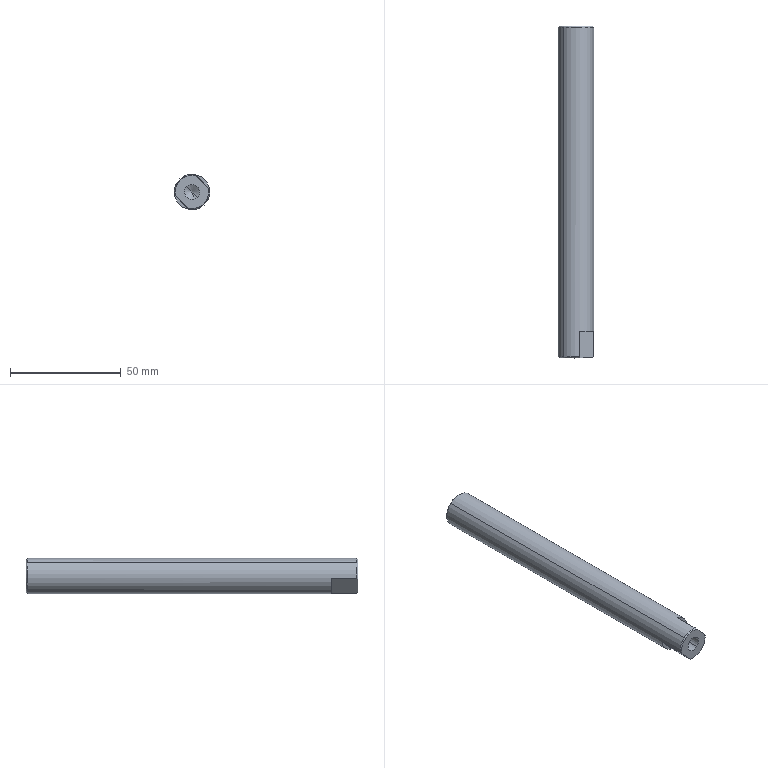Component | SolidWorks | SL021-102-4065.SL4PRT-5 | 1 solid | 21 faces | box 16 x 150 x 16 mm | volume 27965 mm3 | cone 9 | cylinder 6 | plane 6 | commonest cylinder face diameters 6.8 x4 16 x2 | material Bearing Steel
build123d program:
from build123d import *

# Parameters (mm, degrees)
SKETCH1_R           = 8
BOSS_EXTRUDE1_DEPTH = 75
CHAMFER1_SIZE       = 0.5
SKETCH4_OUTSIDE_W   = 48.34
SKETCH4_OUTSIDE_H   = 48.34
SKETCH4_OUTSIDE_W_2 = 13
SKETCH4_OUTSIDE_H_2 = 21.2
CUT_EXTRUDE1_DEPTH  = 12


with BuildPart() as part:
    # Sketch1 → Boss-Extrude1 (new, symmetric)
    with BuildSketch(Plane(origin=(0, 0, 0), x_dir=(1, 0, 0), z_dir=(0, 1, 0))):
        with Locations(Location((0, 0, 0), (0, 0, 270))):
            Circle(SKETCH1_R)
    extrude(amount=BOSS_EXTRUDE1_DEPTH, both=True)

    # Chamfer1
    chamfer1_edges = [part.edges().sort_by_distance(p)[0] for p in [
        (0, -75, -8),
        (0, 75, -8),
    ]]
    chamfer(chamfer1_edges, length=CHAMFER1_SIZE)

    # Sketch2 → M8 Tapped Hole1 (revolve, cut)
    with BuildSketch(Plane(origin=(0, 75, 0), x_dir=(0, 0, 1), z_dir=(1, 0, 0))):
        Polygon((0, 0), (0, 28.293), (3.4, 26.25), (3.4, 0), align=None)
    m8_tapped_hole1 = revolve(axis=Axis((0, 81.35, 0), (0, -1, 0)), mode=Mode.SUBTRACT)

    # Mirror1: M8 Tapped Hole1 across plane
    add(m8_tapped_hole1.mirror(Plane.ZX), mode=Mode.SUBTRACT)

    # Sketch4 outside → Cut-Extrude1 (cut)
    with BuildSketch(Plane.XZ.offset(75)):
        Rectangle(SKETCH4_OUTSIDE_W, SKETCH4_OUTSIDE_H)
        Rectangle(SKETCH4_OUTSIDE_W_2, SKETCH4_OUTSIDE_H_2, mode=Mode.SUBTRACT)
    extrude(amount=-CUT_EXTRUDE1_DEPTH, mode=Mode.SUBTRACT)


solid = part.part

# Placed as in the assembly
solid = solid.moved(Location((-126.163, -15.499, -306.378), (180, 42.687, -180)))
STEP:
#1=COLOUR_RGB('',0.7922,0.8196,0.9333);
#2=FILL_AREA_STYLE_COLOUR('',#1);
#3=FILL_AREA_STYLE('',(#2));
#4=SURFACE_STYLE_FILL_AREA(#3);
#5=SURFACE_SIDE_STYLE('',(#4));
#6=SURFACE_STYLE_USAGE(.BOTH.,#5);
#7=PRESENTATION_STYLE_ASSIGNMENT((#6));
#8=CARTESIAN_POINT('',(-4.876,-2.529,-12.161));
#9=VERTEX_POINT('',#8);
#10=CARTESIAN_POINT('',(-5.058,-2.529,-11.964));
#11=VERTEX_POINT('',#10);
#12=CARTESIAN_POINT('',(-4.967,-2.529,-12.062));
#13=DIRECTION('',(0.,-1.,0.));
#14=DIRECTION('',(-0.678,0.,0.7351));
#15=AXIS2_PLACEMENT_3D('',#12,#13,#14);
#16=CIRCLE('',#15,0.1339);
#17=EDGE_CURVE('',#9,#11,#16,.T.);
#18=ORIENTED_EDGE('',*,*,#17,.F.);
#19=CARTESIAN_POINT('',(-4.876,-3.563,-12.161));
#20=VERTEX_POINT('',#19);
#21=CARTESIAN_POINT('',(-4.876,-3.563,-12.161));
#22=DIRECTION('',(0.,-1.,0.));
#23=VECTOR('',#22,39.37);
#24=LINE('',#21,#23);
#25=EDGE_CURVE('',#9,#20,#24,.T.);
#26=ORIENTED_EDGE('',*,*,#25,.T.);
#27=CARTESIAN_POINT('',(-5.058,-3.563,-11.964));
#28=VERTEX_POINT('',#27);
#29=CARTESIAN_POINT('',(-4.967,-3.563,-12.062));
#30=DIRECTION('',(0.,-1.,0.));
#31=DIRECTION('',(-0.678,0.,0.7351));
#32=AXIS2_PLACEMENT_3D('',#29,#30,#31);
#33=CIRCLE('',#32,0.1339);
#34=EDGE_CURVE('',#20,#28,#33,.T.);
#35=ORIENTED_EDGE('',*,*,#34,.T.);
#36=CARTESIAN_POINT('',(-5.058,-3.563,-11.964));
#37=DIRECTION('',(0.,-1.,0.));
#38=VECTOR('',#37,39.37);
#39=LINE('',#36,#38);
#40=EDGE_CURVE('',#11,#28,#39,.T.);
#41=ORIENTED_EDGE('',*,*,#40,.F.);
#42=EDGE_LOOP('',(#18,#26,#35,#41));
#43=FACE_OUTER_BOUND('',#42,.T.);
#44=CARTESIAN_POINT('',(-4.967,-3.563,-12.062));
#45=DIRECTION('',(0.,-1.,0.));
#46=DIRECTION('',(-0.678,0.,0.7351));
#47=AXIS2_PLACEMENT_3D('',#44,#45,#46);
#48=CYLINDRICAL_SURFACE('',#47,0.1339);
#49=ADVANCED_FACE('',(#43),#48,.F.);
#50=CARTESIAN_POINT('',(-4.967,-2.449,-12.062));
#51=VERTEX_POINT('',#50);
#52=CARTESIAN_POINT('',(-5.058,-2.529,-11.964));
#53=DIRECTION('',(-0.5811,-0.515,0.6301));
#54=VECTOR('',#53,39.37);
#55=LINE('',#52,#54);
#56=EDGE_CURVE('',#51,#11,#55,.T.);
#57=ORIENTED_EDGE('',*,*,#56,.F.);
#58=CARTESIAN_POINT('',(-4.876,-2.529,-12.161));
#59=DIRECTION('',(0.5811,-0.515,-0.6301));
#60=VECTOR('',#59,39.37);
#61=LINE('',#58,#60);
#62=EDGE_CURVE('',#51,#9,#61,.T.);
#63=ORIENTED_EDGE('',*,*,#62,.T.);
#64=ORIENTED_EDGE('',*,*,#17,.T.);
#65=EDGE_LOOP('',(#57,#63,#64));
#66=FACE_OUTER_BOUND('',#65,.T.);
#67=CARTESIAN_POINT('',(-4.967,-2.529,-12.062));
#68=DIRECTION('',(0.,-1.,0.));
#69=DIRECTION('',(-0.678,0.,0.7351));
#70=AXIS2_PLACEMENT_3D('',#67,#68,#69);
#71=CONICAL_SURFACE('',#70,0.1339,1.03);
#72=ADVANCED_FACE('',(#66),#71,.F.);
#73=CARTESIAN_POINT('',(-5.058,1.309,-11.964));
#74=VERTEX_POINT('',#73);
#75=CARTESIAN_POINT('',(-4.876,1.309,-12.161));
#76=VERTEX_POINT('',#75);
#77=CARTESIAN_POINT('',(-4.967,1.309,-12.062));
#78=DIRECTION('',(-0.,1.,-0.));
#79=DIRECTION('',(0.678,0.,-0.7351));
#80=AXIS2_PLACEMENT_3D('',#77,#78,#79);
#81=CIRCLE('',#80,0.1339);
#82=EDGE_CURVE('',#74,#76,#81,.T.);
#83=ORIENTED_EDGE('',*,*,#82,.F.);
#84=CARTESIAN_POINT('',(-5.058,2.343,-11.964));
#85=VERTEX_POINT('',#84);
#86=CARTESIAN_POINT('',(-5.058,2.343,-11.964));
#87=DIRECTION('',(-0.,1.,-0.));
#88=VECTOR('',#87,39.37);
#89=LINE('',#86,#88);
#90=EDGE_CURVE('',#74,#85,#89,.T.);
#91=ORIENTED_EDGE('',*,*,#90,.T.);
#92=CARTESIAN_POINT('',(-4.876,2.343,-12.161));
#93=VERTEX_POINT('',#92);
#94=CARTESIAN_POINT('',(-4.967,2.343,-12.062));
#95=DIRECTION('',(-0.,1.,-0.));
#96=DIRECTION('',(0.678,0.,-0.7351));
#97=AXIS2_PLACEMENT_3D('',#94,#95,#96);
#98=CIRCLE('',#97,0.1339);
#99=EDGE_CURVE('',#85,#93,#98,.T.);
#100=ORIENTED_EDGE('',*,*,#99,.T.);
#101=CARTESIAN_POINT('',(-4.876,2.343,-12.161));
#102=DIRECTION('',(-0.,1.,-0.));
#103=VECTOR('',#102,39.37);
#104=LINE('',#101,#103);
#105=EDGE_CURVE('',#76,#93,#104,.T.);
#106=ORIENTED_EDGE('',*,*,#105,.F.);
#107=EDGE_LOOP('',(#83,#91,#100,#106));
#108=FACE_OUTER_BOUND('',#107,.T.);
#109=CARTESIAN_POINT('',(-4.967,2.343,-12.062));
#110=DIRECTION('',(-0.,1.,-0.));
#111=DIRECTION('',(0.678,0.,-0.7351));
#112=AXIS2_PLACEMENT_3D('',#109,#110,#111);
#113=CYLINDRICAL_SURFACE('',#112,0.1339);
#114=ADVANCED_FACE('',(#108),#113,.F.);
#115=CARTESIAN_POINT('',(-4.967,1.229,-12.062));
#116=VERTEX_POINT('',#115);
#117=CARTESIAN_POINT('',(-4.876,1.309,-12.161));
#118=DIRECTION('',(0.5811,0.515,-0.6301));
#119=VECTOR('',#118,39.37);
#120=LINE('',#117,#119);
#121=EDGE_CURVE('',#116,#76,#120,.T.);
#122=ORIENTED_EDGE('',*,*,#121,.F.);
#123=CARTESIAN_POINT('',(-5.058,1.309,-11.964));
#124=DIRECTION('',(-0.5811,0.515,0.6301));
#125=VECTOR('',#124,39.37);
#126=LINE('',#123,#125);
#127=EDGE_CURVE('',#116,#74,#126,.T.);
#128=ORIENTED_EDGE('',*,*,#127,.T.);
#129=ORIENTED_EDGE('',*,*,#82,.T.);
#130=EDGE_LOOP('',(#122,#128,#129));
#131=FACE_OUTER_BOUND('',#130,.T.);
#132=CARTESIAN_POINT('',(-4.967,1.309,-12.062));
#133=DIRECTION('',(-0.,1.,-0.));
#134=DIRECTION('',(0.678,0.,-0.7351));
#135=AXIS2_PLACEMENT_3D('',#132,#133,#134);
#136=CONICAL_SURFACE('',#135,0.1339,1.03);
#137=ADVANCED_FACE('',(#131),#136,.F.);
#138=CARTESIAN_POINT('',(-4.767,2.343,-12.279));
#139=VERTEX_POINT('',#138);
#140=CARTESIAN_POINT('',(-5.167,2.343,-11.845));
#141=VERTEX_POINT('',#140);
#142=CARTESIAN_POINT('',(-4.967,2.343,-12.062));
#143=DIRECTION('',(-0.,1.,-0.));
#144=DIRECTION('',(0.678,0.,-0.7351));
#145=AXIS2_PLACEMENT_3D('',#142,#143,#144);
#146=CIRCLE('',#145,0.2953);
#147=EDGE_CURVE('',#139,#141,#146,.T.);
#148=ORIENTED_EDGE('',*,*,#147,.F.);
#149=CARTESIAN_POINT('',(-4.754,2.323,-12.294));
#150=VERTEX_POINT('',#149);
#151=CARTESIAN_POINT('',(-4.767,2.343,-12.279));
#152=DIRECTION('',(0.4794,-0.7071,-0.5198));
#153=VECTOR('',#152,39.37);
#154=LINE('',#151,#153);
#155=EDGE_CURVE('',#139,#150,#154,.T.);
#156=ORIENTED_EDGE('',*,*,#155,.T.);
#157=CARTESIAN_POINT('',(-5.181,2.323,-11.831));
#158=VERTEX_POINT('',#157);
#159=CARTESIAN_POINT('',(-4.967,2.323,-12.062));
#160=DIRECTION('',(0.,-1.,0.));
#161=DIRECTION('',(0.678,0.,-0.7351));
#162=AXIS2_PLACEMENT_3D('',#159,#160,#161);
#163=CIRCLE('',#162,0.315);
#164=EDGE_CURVE('',#158,#150,#163,.T.);
#165=ORIENTED_EDGE('',*,*,#164,.F.);
#166=CARTESIAN_POINT('',(-5.167,2.343,-11.845));
#167=DIRECTION('',(-0.4794,-0.7071,0.5198));
#168=VECTOR('',#167,39.37);
#169=LINE('',#166,#168);
#170=EDGE_CURVE('',#141,#158,#169,.T.);
#171=ORIENTED_EDGE('',*,*,#170,.F.);
#172=EDGE_LOOP('',(#148,#156,#165,#171));
#173=FACE_OUTER_BOUND('',#172,.T.);
#174=CARTESIAN_POINT('',(-4.967,2.343,-12.062));
#175=DIRECTION('',(0.,-1.,0.));
#176=DIRECTION('',(-0.678,0.,0.7351));
#177=AXIS2_PLACEMENT_3D('',#174,#175,#176);
#178=CONICAL_SURFACE('',#177,0.2953,0.7854);
#179=ADVANCED_FACE('',(#173),#178,.T.);
#180=CARTESIAN_POINT('',(-4.767,-3.563,-12.279));
#181=VERTEX_POINT('',#180);
#182=CARTESIAN_POINT('',(-4.679,-3.563,-11.997));
#183=VERTEX_POINT('',#182);
#184=CARTESIAN_POINT('',(-4.967,-3.563,-12.062));
#185=DIRECTION('',(0.,-1.,0.));
#186=DIRECTION('',(0.678,0.,-0.7351));
#187=AXIS2_PLACEMENT_3D('',#184,#185,#186);
#188=CIRCLE('',#187,0.2953);
#189=EDGE_CURVE('',#181,#183,#188,.T.);
#190=ORIENTED_EDGE('',*,*,#189,.F.);
#191=CARTESIAN_POINT('',(-4.754,-3.543,-12.294));
#192=VERTEX_POINT('',#191);
#193=CARTESIAN_POINT('',(-4.754,-3.543,-12.294));
#194=DIRECTION('',(0.4794,0.7071,-0.5198));
#195=VECTOR('',#194,39.37);
#196=LINE('',#193,#195);
#197=EDGE_CURVE('',#181,#192,#196,.T.);
#198=ORIENTED_EDGE('',*,*,#197,.T.);
#199=CARTESIAN_POINT('',(-4.654,-3.543,-12.024));
#200=VERTEX_POINT('',#199);
#201=CARTESIAN_POINT('',(-4.967,-3.543,-12.062));
#202=DIRECTION('',(-0.,1.,-0.));
#203=DIRECTION('',(0.678,0.,-0.7351));
#204=AXIS2_PLACEMENT_3D('',#201,#202,#203);
#205=CIRCLE('',#204,0.315);
#206=EDGE_CURVE('',#200,#192,#205,.T.);
#207=ORIENTED_EDGE('',*,*,#206,.F.);
#208=CARTESIAN_POINT('',(-4.654,-3.543,-12.024));
#209=CARTESIAN_POINT('',(-4.663,-3.55,-12.015));
#210=CARTESIAN_POINT('',(-4.671,-3.557,-12.006));
#211=CARTESIAN_POINT('',(-4.679,-3.563,-11.997));
#212=B_SPLINE_CURVE_WITH_KNOTS('',3,(#208,#209,#210,#211),.UNSPECIFIED.,.F.,.F.,(4,4),(0.01516,0.01621),.UNSPECIFIED.);
#213=EDGE_CURVE('',#200,#183,#212,.T.);
#214=ORIENTED_EDGE('',*,*,#213,.T.);
#215=EDGE_LOOP('',(#190,#198,#207,#214));
#216=FACE_OUTER_BOUND('',#215,.T.);
#217=CARTESIAN_POINT('',(-4.967,-3.543,-12.062));
#218=DIRECTION('',(-0.,1.,-0.));
#219=DIRECTION('',(0.678,0.,-0.7351));
#220=AXIS2_PLACEMENT_3D('',#217,#218,#219);
#221=CONICAL_SURFACE('',#220,0.315,0.7854);
#222=ADVANCED_FACE('',(#216),#221,.T.);
#223=ORIENTED_EDGE('',*,*,#164,.T.);
#224=CARTESIAN_POINT('',(-4.754,2.343,-12.294));
#225=DIRECTION('',(0.,-1.,0.));
#226=VECTOR('',#225,39.37);
#227=LINE('',#224,#226);
#228=EDGE_CURVE('',#150,#192,#227,.T.);
#229=ORIENTED_EDGE('',*,*,#228,.T.);
#230=CARTESIAN_POINT('',(-5.031,-3.543,-12.371));
#231=VERTEX_POINT('',#230);
#232=CARTESIAN_POINT('',(-4.967,-3.543,-12.062));
#233=DIRECTION('',(-0.,1.,-0.));
#234=DIRECTION('',(0.678,0.,-0.7351));
#235=AXIS2_PLACEMENT_3D('',#232,#233,#234);
#236=CIRCLE('',#235,0.315);
#237=EDGE_CURVE('',#192,#231,#236,.T.);
#238=ORIENTED_EDGE('',*,*,#237,.T.);
#239=CARTESIAN_POINT('',(-5.031,-3.091,-12.371));
#240=VERTEX_POINT('',#239);
#241=CARTESIAN_POINT('',(-5.031,2.343,-12.371));
#242=DIRECTION('',(0.,-1.,0.));
#243=VECTOR('',#242,39.37);
#244=LINE('',#241,#243);
#245=EDGE_CURVE('',#240,#231,#244,.T.);
#246=ORIENTED_EDGE('',*,*,#245,.F.);
#247=CARTESIAN_POINT('',(-5.28,-3.091,-12.101));
#248=VERTEX_POINT('',#247);
#249=CARTESIAN_POINT('',(-4.967,-3.091,-12.062));
#250=DIRECTION('',(0.,-1.,0.));
#251=DIRECTION('',(-0.678,0.,0.7351));
#252=AXIS2_PLACEMENT_3D('',#249,#250,#251);
#253=CIRCLE('',#252,0.315);
#254=EDGE_CURVE('',#248,#240,#253,.T.);
#255=ORIENTED_EDGE('',*,*,#254,.F.);
#256=CARTESIAN_POINT('',(-5.28,-3.543,-12.101));
#257=VERTEX_POINT('',#256);
#258=CARTESIAN_POINT('',(-5.28,2.343,-12.101));
#259=DIRECTION('',(-0.,1.,-0.));
#260=VECTOR('',#259,39.37);
#261=LINE('',#258,#260);
#262=EDGE_CURVE('',#257,#248,#261,.T.);
#263=ORIENTED_EDGE('',*,*,#262,.F.);
#264=CARTESIAN_POINT('',(-5.181,-3.543,-11.831));
#265=VERTEX_POINT('',#264);
#266=CARTESIAN_POINT('',(-4.967,-3.543,-12.062));
#267=DIRECTION('',(-0.,1.,-0.));
#268=DIRECTION('',(0.678,0.,-0.7351));
#269=AXIS2_PLACEMENT_3D('',#266,#267,#268);
#270=CIRCLE('',#269,0.315);
#271=EDGE_CURVE('',#257,#265,#270,.T.);
#272=ORIENTED_EDGE('',*,*,#271,.T.);
#273=CARTESIAN_POINT('',(-5.181,2.343,-11.831));
#274=DIRECTION('',(0.,-1.,0.));
#275=VECTOR('',#274,39.37);
#276=LINE('',#273,#275);
#277=EDGE_CURVE('',#158,#265,#276,.T.);
#278=ORIENTED_EDGE('',*,*,#277,.F.);
#279=EDGE_LOOP('',(#223,#229,#238,#246,#255,#263,#272,#278));
#280=FACE_OUTER_BOUND('',#279,.T.);
#281=CARTESIAN_POINT('',(-4.967,2.343,-12.062));
#282=DIRECTION('',(0.,-1.,0.));
#283=DIRECTION('',(-0.678,0.,0.7351));
#284=AXIS2_PLACEMENT_3D('',#281,#282,#283);
#285=CYLINDRICAL_SURFACE('',#284,0.315);
#286=ADVANCED_FACE('',(#280),#285,.T.);
#287=ORIENTED_EDGE('',*,*,#228,.F.);
#288=CARTESIAN_POINT('',(-4.967,2.323,-12.062));
#289=DIRECTION('',(0.,-1.,0.));
#290=DIRECTION('',(0.678,0.,-0.7351));
#291=AXIS2_PLACEMENT_3D('',#288,#289,#290);
#292=CIRCLE('',#291,0.315);
#293=EDGE_CURVE('',#150,#158,#292,.T.);
#294=ORIENTED_EDGE('',*,*,#293,.T.);
#295=ORIENTED_EDGE('',*,*,#277,.T.);
#296=CARTESIAN_POINT('',(-4.903,-3.543,-11.754));
#297=VERTEX_POINT('',#296);
#298=CARTESIAN_POINT('',(-4.967,-3.543,-12.062));
#299=DIRECTION('',(-0.,1.,-0.));
#300=DIRECTION('',(0.678,0.,-0.7351));
#301=AXIS2_PLACEMENT_3D('',#298,#299,#300);
#302=CIRCLE('',#301,0.315);
#303=EDGE_CURVE('',#265,#297,#302,.T.);
#304=ORIENTED_EDGE('',*,*,#303,.T.);
#305=CARTESIAN_POINT('',(-4.903,-3.091,-11.754));
#306=VERTEX_POINT('',#305);
#307=CARTESIAN_POINT('',(-4.903,2.343,-11.754));
#308=DIRECTION('',(0.,-1.,0.));
#309=VECTOR('',#308,39.37);
#310=LINE('',#307,#309);
#311=EDGE_CURVE('',#306,#297,#310,.T.);
#312=ORIENTED_EDGE('',*,*,#311,.F.);
#313=CARTESIAN_POINT('',(-4.654,-3.091,-12.024));
#314=VERTEX_POINT('',#313);
#315=CARTESIAN_POINT('',(-4.967,-3.091,-12.062));
#316=DIRECTION('',(0.,-1.,0.));
#317=DIRECTION('',(-0.678,0.,0.7351));
#318=AXIS2_PLACEMENT_3D('',#315,#316,#317);
#319=CIRCLE('',#318,0.315);
#320=EDGE_CURVE('',#314,#306,#319,.T.);
#321=ORIENTED_EDGE('',*,*,#320,.F.);
#322=CARTESIAN_POINT('',(-4.654,2.343,-12.024));
#323=DIRECTION('',(-0.,1.,-0.));
#324=VECTOR('',#323,39.37);
#325=LINE('',#322,#324);
#326=EDGE_CURVE('',#200,#314,#325,.T.);
#327=ORIENTED_EDGE('',*,*,#326,.F.);
#328=ORIENTED_EDGE('',*,*,#206,.T.);
#329=EDGE_LOOP('',(#287,#294,#295,#304,#312,#321,#327,#328));
#330=FACE_OUTER_BOUND('',#329,.T.);
#331=CARTESIAN_POINT('',(-4.967,2.343,-12.062));
#332=DIRECTION('',(0.,-1.,0.));
#333=DIRECTION('',(-0.678,0.,0.7351));
#334=AXIS2_PLACEMENT_3D('',#331,#332,#333);
#335=CYLINDRICAL_SURFACE('',#334,0.315);
#336=ADVANCED_FACE('',(#330),#335,.T.);
#337=CARTESIAN_POINT('',(-4.967,-3.563,-12.062));
#338=DIRECTION('',(0.,-1.,0.));
#339=DIRECTION('',(-0.678,0.,0.7351));
#340=AXIS2_PLACEMENT_3D('',#337,#338,#339);
#341=CIRCLE('',#340,0.1339);
#342=EDGE_CURVE('',#28,#20,#341,.T.);
#343=ORIENTED_EDGE('',*,*,#342,.F.);
#344=ORIENTED_EDGE('',*,*,#34,.F.);
#345=EDGE_LOOP('',(#343,#344));
#346=FACE_BOUND('',#345,.T.);
#347=CARTESIAN_POINT('',(-5.255,-3.563,-12.127));
#348=VERTEX_POINT('',#347);
#349=CARTESIAN_POINT('',(-5.055,-3.563,-12.344));
#350=VERTEX_POINT('',#349);
#351=CARTESIAN_POINT('',(-5.438,-3.563,-11.929));
#352=DIRECTION('',(0.678,-0.,-0.7351));
#353=VECTOR('',#352,39.37);
#354=LINE('',#351,#353);
#355=EDGE_CURVE('',#348,#350,#354,.T.);
#356=ORIENTED_EDGE('',*,*,#355,.T.);
#357=CARTESIAN_POINT('',(-4.967,-3.563,-12.062));
#358=DIRECTION('',(0.,-1.,0.));
#359=DIRECTION('',(0.678,0.,-0.7351));
#360=AXIS2_PLACEMENT_3D('',#357,#358,#359);
#361=CIRCLE('',#360,0.2953);
#362=EDGE_CURVE('',#350,#181,#361,.T.);
#363=ORIENTED_EDGE('',*,*,#362,.T.);
#364=ORIENTED_EDGE('',*,*,#189,.T.);
#365=CARTESIAN_POINT('',(-4.879,-3.563,-11.78));
#366=VERTEX_POINT('',#365);
#367=CARTESIAN_POINT('',(-5.062,-3.563,-11.582));
#368=DIRECTION('',(-0.678,0.,0.7351));
#369=VECTOR('',#368,39.37);
#370=LINE('',#367,#369);
#371=EDGE_CURVE('',#183,#366,#370,.T.);
#372=ORIENTED_EDGE('',*,*,#371,.T.);
#373=CARTESIAN_POINT('',(-4.967,-3.563,-12.062));
#374=DIRECTION('',(0.,-1.,0.));
#375=DIRECTION('',(0.678,0.,-0.7351));
#376=AXIS2_PLACEMENT_3D('',#373,#374,#375);
#377=CIRCLE('',#376,0.2953);
#378=EDGE_CURVE('',#366,#348,#377,.T.);
#379=ORIENTED_EDGE('',*,*,#378,.T.);
#380=EDGE_LOOP('',(#356,#363,#364,#372,#379));
#381=FACE_OUTER_BOUND('',#380,.T.);
#382=CARTESIAN_POINT('',(-4.967,-3.563,-12.062));
#383=DIRECTION('',(-0.,1.,-0.));
#384=DIRECTION('',(0.678,-0.,-0.7351));
#385=AXIS2_PLACEMENT_3D('',#382,#383,#384);
#386=PLANE('',#385);
#387=ADVANCED_FACE('',(#346,#381),#386,.F.);
#388=ORIENTED_EDGE('',*,*,#271,.F.);
#389=CARTESIAN_POINT('',(-5.28,-3.543,-12.101));
#390=CARTESIAN_POINT('',(-5.272,-3.55,-12.109));
#391=CARTESIAN_POINT('',(-5.263,-3.557,-12.118));
#392=CARTESIAN_POINT('',(-5.255,-3.563,-12.127));
#393=B_SPLINE_CURVE_WITH_KNOTS('',3,(#389,#390,#391,#392),.UNSPECIFIED.,.F.,.F.,(4,4),(0.01516,0.01621),.UNSPECIFIED.);
#394=EDGE_CURVE('',#257,#348,#393,.T.);
#395=ORIENTED_EDGE('',*,*,#394,.T.);
#396=ORIENTED_EDGE('',*,*,#378,.F.);
#397=CARTESIAN_POINT('',(-4.879,-3.563,-11.78));
#398=CARTESIAN_POINT('',(-4.887,-3.557,-11.771));
#399=CARTESIAN_POINT('',(-4.895,-3.55,-11.762));
#400=CARTESIAN_POINT('',(-4.903,-3.543,-11.754));
#401=B_SPLINE_CURVE_WITH_KNOTS('',3,(#397,#398,#399,#400),.UNSPECIFIED.,.F.,.F.,(4,4),(0.02403,0.02509),.UNSPECIFIED.);
#402=EDGE_CURVE('',#366,#297,#401,.T.);
#403=ORIENTED_EDGE('',*,*,#402,.T.);
#404=ORIENTED_EDGE('',*,*,#303,.F.);
#405=EDGE_LOOP('',(#388,#395,#396,#403,#404));
#406=FACE_OUTER_BOUND('',#405,.T.);
#407=CARTESIAN_POINT('',(-4.967,-3.543,-12.062));
#408=DIRECTION('',(-0.,1.,-0.));
#409=DIRECTION('',(0.678,0.,-0.7351));
#410=AXIS2_PLACEMENT_3D('',#407,#408,#409);
#411=CONICAL_SURFACE('',#410,0.315,0.7854);
#412=ADVANCED_FACE('',(#406),#411,.T.);
#413=ORIENTED_EDGE('',*,*,#197,.F.);
#414=ORIENTED_EDGE('',*,*,#362,.F.);
#415=CARTESIAN_POINT('',(-5.055,-3.563,-12.344));
#416=CARTESIAN_POINT('',(-5.047,-3.557,-12.353));
#417=CARTESIAN_POINT('',(-5.039,-3.55,-12.362));
#418=CARTESIAN_POINT('',(-5.031,-3.543,-12.371));
#419=B_SPLINE_CURVE_WITH_KNOTS('',3,(#415,#416,#417,#418),.UNSPECIFIED.,.F.,.F.,(4,4),(0.02403,0.02509),.UNSPECIFIED.);
#420=EDGE_CURVE('',#350,#231,#419,.T.);
#421=ORIENTED_EDGE('',*,*,#420,.T.);
#422=ORIENTED_EDGE('',*,*,#237,.F.);
#423=EDGE_LOOP('',(#413,#414,#421,#422));
#424=FACE_OUTER_BOUND('',#423,.T.);
#425=CARTESIAN_POINT('',(-4.967,-3.543,-12.062));
#426=DIRECTION('',(-0.,1.,-0.));
#427=DIRECTION('',(0.678,0.,-0.7351));
#428=AXIS2_PLACEMENT_3D('',#425,#426,#427);
#429=CONICAL_SURFACE('',#428,0.315,0.7854);
#430=ADVANCED_FACE('',(#424),#429,.T.);
#431=CARTESIAN_POINT('',(-4.967,2.343,-12.062));
#432=DIRECTION('',(-0.,1.,-0.));
#433=DIRECTION('',(0.678,0.,-0.7351));
#434=AXIS2_PLACEMENT_3D('',#431,#432,#433);
#435=CIRCLE('',#434,0.1339);
#436=EDGE_CURVE('',#93,#85,#435,.T.);
#437=ORIENTED_EDGE('',*,*,#436,.F.);
#438=ORIENTED_EDGE('',*,*,#99,.F.);
#439=EDGE_LOOP('',(#437,#438));
#440=FACE_BOUND('',#439,.T.);
#441=CARTESIAN_POINT('',(-4.967,2.343,-12.062));
#442=DIRECTION('',(-0.,1.,-0.));
#443=DIRECTION('',(0.678,0.,-0.7351));
#444=AXIS2_PLACEMENT_3D('',#441,#442,#443);
#445=CIRCLE('',#444,0.2953);
#446=EDGE_CURVE('',#141,#139,#445,.T.);
#447=ORIENTED_EDGE('',*,*,#446,.T.);
#448=ORIENTED_EDGE('',*,*,#147,.T.);
#449=EDGE_LOOP('',(#447,#448));
#450=FACE_OUTER_BOUND('',#449,.T.);
#451=CARTESIAN_POINT('',(-4.967,2.343,-12.062));
#452=DIRECTION('',(-0.,1.,-0.));
#453=DIRECTION('',(0.678,-0.,-0.7351));
#454=AXIS2_PLACEMENT_3D('',#451,#452,#453);
#455=PLANE('',#454);
#456=ADVANCED_FACE('',(#440,#450),#455,.T.);
#457=ORIENTED_EDGE('',*,*,#155,.F.);
#458=ORIENTED_EDGE('',*,*,#446,.F.);
#459=ORIENTED_EDGE('',*,*,#170,.T.);
#460=ORIENTED_EDGE('',*,*,#293,.F.);
#461=EDGE_LOOP('',(#457,#458,#459,#460));
#462=FACE_OUTER_BOUND('',#461,.T.);
#463=CARTESIAN_POINT('',(-4.967,2.343,-12.062));
#464=DIRECTION('',(0.,-1.,0.));
#465=DIRECTION('',(-0.678,0.,0.7351));
#466=AXIS2_PLACEMENT_3D('',#463,#464,#465);
#467=CONICAL_SURFACE('',#466,0.2953,0.7854);
#468=ADVANCED_FACE('',(#462),#467,.T.);
#469=ORIENTED_EDGE('',*,*,#127,.F.);
#470=ORIENTED_EDGE('',*,*,#121,.T.);
#471=CARTESIAN_POINT('',(-4.967,1.309,-12.062));
#472=DIRECTION('',(-0.,1.,-0.));
#473=DIRECTION('',(0.678,0.,-0.7351));
#474=AXIS2_PLACEMENT_3D('',#471,#472,#473);
#475=CIRCLE('',#474,0.1339);
#476=EDGE_CURVE('',#76,#74,#475,.T.);
#477=ORIENTED_EDGE('',*,*,#476,.T.);
#478=EDGE_LOOP('',(#469,#470,#477));
#479=FACE_OUTER_BOUND('',#478,.T.);
#480=CARTESIAN_POINT('',(-4.967,1.309,-12.062));
#481=DIRECTION('',(-0.,1.,-0.));
#482=DIRECTION('',(0.678,0.,-0.7351));
#483=AXIS2_PLACEMENT_3D('',#480,#481,#482);
#484=CONICAL_SURFACE('',#483,0.1339,1.03);
#485=ADVANCED_FACE('',(#479),#484,.F.);
#486=ORIENTED_EDGE('',*,*,#90,.F.);
#487=ORIENTED_EDGE('',*,*,#476,.F.);
#488=ORIENTED_EDGE('',*,*,#105,.T.);
#489=ORIENTED_EDGE('',*,*,#436,.T.);
#490=EDGE_LOOP('',(#486,#487,#488,#489));
#491=FACE_OUTER_BOUND('',#490,.T.);
#492=CARTESIAN_POINT('',(-4.967,2.343,-12.062));
#493=DIRECTION('',(-0.,1.,-0.));
#494=DIRECTION('',(0.678,0.,-0.7351));
#495=AXIS2_PLACEMENT_3D('',#492,#493,#494);
#496=CYLINDRICAL_SURFACE('',#495,0.1339);
#497=ADVANCED_FACE('',(#491),#496,.F.);
#498=ORIENTED_EDGE('',*,*,#62,.F.);
#499=ORIENTED_EDGE('',*,*,#56,.T.);
#500=CARTESIAN_POINT('',(-4.967,-2.529,-12.062));
#501=DIRECTION('',(0.,-1.,0.));
#502=DIRECTION('',(-0.678,0.,0.7351));
#503=AXIS2_PLACEMENT_3D('',#500,#501,#502);
#504=CIRCLE('',#503,0.1339);
#505=EDGE_CURVE('',#11,#9,#504,.T.);
#506=ORIENTED_EDGE('',*,*,#505,.T.);
#507=EDGE_LOOP('',(#498,#499,#506));
#508=FACE_OUTER_BOUND('',#507,.T.);
#509=CARTESIAN_POINT('',(-4.967,-2.529,-12.062));
#510=DIRECTION('',(0.,-1.,0.));
#511=DIRECTION('',(-0.678,0.,0.7351));
#512=AXIS2_PLACEMENT_3D('',#509,#510,#511);
#513=CONICAL_SURFACE('',#512,0.1339,1.03);
#514=ADVANCED_FACE('',(#508),#513,.F.);
#515=ORIENTED_EDGE('',*,*,#25,.F.);
#516=ORIENTED_EDGE('',*,*,#505,.F.);
#517=ORIENTED_EDGE('',*,*,#40,.T.);
#518=ORIENTED_EDGE('',*,*,#342,.T.);
#519=EDGE_LOOP('',(#515,#516,#517,#518));
#520=FACE_OUTER_BOUND('',#519,.T.);
#521=CARTESIAN_POINT('',(-4.967,-3.563,-12.062));
#522=DIRECTION('',(0.,-1.,0.));
#523=DIRECTION('',(-0.678,0.,0.7351));
#524=AXIS2_PLACEMENT_3D('',#521,#522,#523);
#525=CYLINDRICAL_SURFACE('',#524,0.1339);
#526=ADVANCED_FACE('',(#520),#525,.F.);
#527=ORIENTED_EDGE('',*,*,#326,.T.);
#528=CARTESIAN_POINT('',(-5.062,-3.091,-11.582));
#529=DIRECTION('',(-0.678,0.,0.7351));
#530=VECTOR('',#529,39.37);
#531=LINE('',#528,#530);
#532=EDGE_CURVE('',#314,#306,#531,.T.);
#533=ORIENTED_EDGE('',*,*,#532,.T.);
#534=ORIENTED_EDGE('',*,*,#311,.T.);
#535=ORIENTED_EDGE('',*,*,#402,.F.);
#536=ORIENTED_EDGE('',*,*,#371,.F.);
#537=ORIENTED_EDGE('',*,*,#213,.F.);
#538=EDGE_LOOP('',(#527,#533,#534,#535,#536,#537));
#539=FACE_OUTER_BOUND('',#538,.T.);
#540=CARTESIAN_POINT('',(-5.062,-3.091,-11.582));
#541=DIRECTION('',(0.7351,0.,0.678));
#542=DIRECTION('',(0.678,-0.,-0.7351));
#543=AXIS2_PLACEMENT_3D('',#540,#541,#542);
#544=PLANE('',#543);
#545=ADVANCED_FACE('',(#539),#544,.T.);
#546=ORIENTED_EDGE('',*,*,#320,.T.);
#547=ORIENTED_EDGE('',*,*,#532,.F.);
#548=EDGE_LOOP('',(#546,#547));
#549=FACE_OUTER_BOUND('',#548,.T.);
#550=CARTESIAN_POINT('',(-4.967,-3.091,-12.062));
#551=DIRECTION('',(0.,-1.,0.));
#552=DIRECTION('',(-0.678,0.,0.7351));
#553=AXIS2_PLACEMENT_3D('',#550,#551,#552);
#554=PLANE('',#553);
#555=ADVANCED_FACE('',(#549),#554,.T.);
#556=ORIENTED_EDGE('',*,*,#254,.T.);
#557=CARTESIAN_POINT('',(-5.438,-3.091,-11.929));
#558=DIRECTION('',(0.678,-0.,-0.7351));
#559=VECTOR('',#558,39.37);
#560=LINE('',#557,#559);
#561=EDGE_CURVE('',#248,#240,#560,.T.);
#562=ORIENTED_EDGE('',*,*,#561,.F.);
#563=EDGE_LOOP('',(#556,#562));
#564=FACE_OUTER_BOUND('',#563,.T.);
#565=CARTESIAN_POINT('',(-4.967,-3.091,-12.062));
#566=DIRECTION('',(0.,-1.,0.));
#567=DIRECTION('',(-0.678,0.,0.7351));
#568=AXIS2_PLACEMENT_3D('',#565,#566,#567);
#569=PLANE('',#568);
#570=ADVANCED_FACE('',(#564),#569,.T.);
#571=ORIENTED_EDGE('',*,*,#262,.T.);
#572=ORIENTED_EDGE('',*,*,#561,.T.);
#573=ORIENTED_EDGE('',*,*,#245,.T.);
#574=ORIENTED_EDGE('',*,*,#420,.F.);
#575=ORIENTED_EDGE('',*,*,#355,.F.);
#576=ORIENTED_EDGE('',*,*,#394,.F.);
#577=EDGE_LOOP('',(#571,#572,#573,#574,#575,#576));
#578=FACE_OUTER_BOUND('',#577,.T.);
#579=CARTESIAN_POINT('',(-5.438,-3.091,-11.929));
#580=DIRECTION('',(-0.7351,-0.,-0.678));
#581=DIRECTION('',(-0.678,0.,0.7351));
#582=AXIS2_PLACEMENT_3D('',#579,#580,#581);
#583=PLANE('',#582);
#584=ADVANCED_FACE('',(#578),#583,.T.);
#585=CLOSED_SHELL('',(#49,#72,#114,#137,#179,#222,#286,#336,#387,#412,#430,#456,#468,#485,#497,#514,#526,#545,#555,#570,#584));
#586=MANIFOLD_SOLID_BREP('',#585);
#587=STYLED_ITEM('',(#7),#586);
#588=(LENGTH_UNIT()NAMED_UNIT(*)SI_UNIT($,.METRE.));
#589=LENGTH_MEASURE_WITH_UNIT(LENGTH_MEASURE(0.0254),#588);
#590=DIMENSIONAL_EXPONENTS(1.,0.,0.,0.,0.,0.,0.);
#591=(CONVERSION_BASED_UNIT('',#589)LENGTH_UNIT()NAMED_UNIT(#590));
#592=UNCERTAINTY_MEASURE_WITH_UNIT(LENGTH_MEASURE(0.00001),#591,'','');
#593=(NAMED_UNIT(*)PLANE_ANGLE_UNIT()SI_UNIT($,.RADIAN.));
#594=(NAMED_UNIT(*)SI_UNIT($,.STERADIAN.)SOLID_ANGLE_UNIT());
#595=(GEOMETRIC_REPRESENTATION_CONTEXT(3)GLOBAL_UNCERTAINTY_ASSIGNED_CONTEXT((#592))GLOBAL_UNIT_ASSIGNED_CONTEXT((#591,#593,#594))REPRESENTATION_CONTEXT('',''));
#596=MECHANICAL_DESIGN_GEOMETRIC_PRESENTATION_REPRESENTATION('',(#587),#595);
#597=PRESENTATION_LAYER_ASSIGNMENT('','',(#587));
#598=CARTESIAN_POINT('',(0.,0.,0.));
#599=DIRECTION('',(0.,0.,1.));
#600=DIRECTION('',(1.,0.,0.));
#601=AXIS2_PLACEMENT_3D('',#598,#599,#600);
#602=(LENGTH_UNIT()NAMED_UNIT(*)SI_UNIT($,.METRE.));
#603=LENGTH_MEASURE_WITH_UNIT(LENGTH_MEASURE(0.0254),#602);
#604=DIMENSIONAL_EXPONENTS(1.,0.,0.,0.,0.,0.,0.);
#605=(CONVERSION_BASED_UNIT('',#603)LENGTH_UNIT()NAMED_UNIT(#604));
#606=UNCERTAINTY_MEASURE_WITH_UNIT(LENGTH_MEASURE(0.00001),#605,'','');
#607=(NAMED_UNIT(*)PLANE_ANGLE_UNIT()SI_UNIT($,.RADIAN.));
#608=(NAMED_UNIT(*)SI_UNIT($,.STERADIAN.)SOLID_ANGLE_UNIT());
#609=(GEOMETRIC_REPRESENTATION_CONTEXT(3)GLOBAL_UNCERTAINTY_ASSIGNED_CONTEXT((#606))GLOBAL_UNIT_ASSIGNED_CONTEXT((#605,#607,#608))REPRESENTATION_CONTEXT('',''));
#610=ADVANCED_BREP_SHAPE_REPRESENTATION('',(#586,#601),#609);